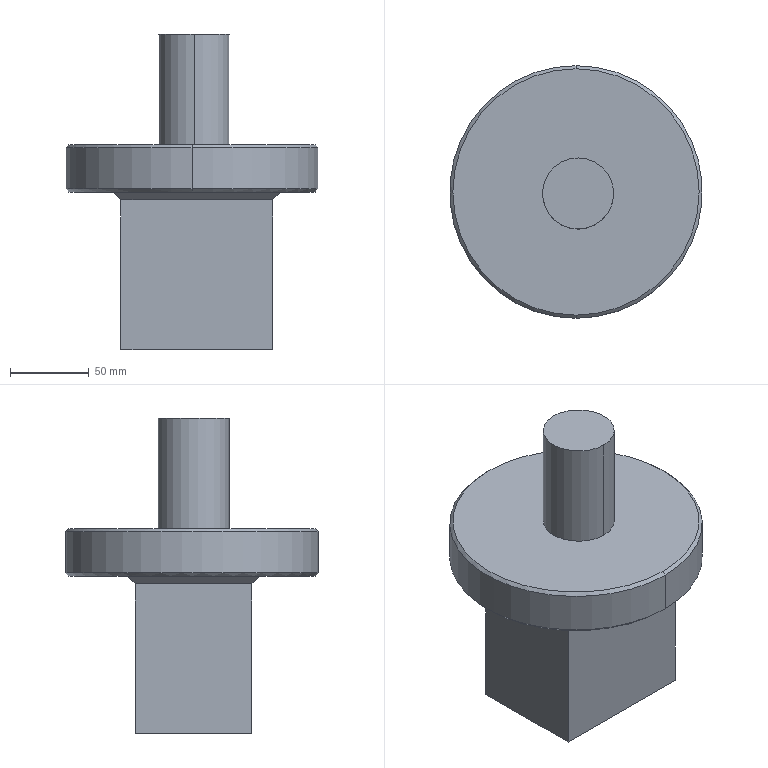Component | SolidWorks | PressureHead-1 | 1 solid | 20 faces | box 160 x 160 x 200 mm | volume 1427339 mm3 | plane 12 | cone 4 | cylinder 4 | commonest cylinder face diameters 45 x2 160 x2
build123d program:
from build123d import *

# Parameters (mm, degrees)
SKETCH1_W           = 80
SKETCH1_H           = 30
SKETCH2_W           = 74
SKETCH2_H           = 96
BOSS_EXTRUDE1_DEPTH = 100
SKETCH3_W           = 22.5
SKETCH3_H           = 70
CHAMFER1_SIZE2      = 2
CHAMFER1_SIZE       = 2
CHAMFER2_SIZE       = 5


with BuildPart() as part:
    # Sketch1 → Revolve1 (revolve)
    with BuildSketch(Plane.XZ.offset(1.405), mode=Mode.PRIVATE) as revolve1_sk:
        with Locations((41.055, 15)):
            Rectangle(SKETCH1_W, SKETCH1_H)
    revolve(revolve1_sk.sketch.rotate(Axis((1.055, -1.405, 30), (0, 0, -1)), 180), axis=Axis((1.055, -1.405, 30), (0, 0, -1)))

    # Sketch2 → Boss-Extrude1 (add)
    with BuildSketch(Plane.XY.offset(30)):
        with Locations((0.05486, 1.595)):
            Rectangle(SKETCH2_W, SKETCH2_H)
    extrude(amount=BOSS_EXTRUDE1_DEPTH)

    # Sketch3 → Revolve2 (revolve)
    with BuildSketch(Plane.XZ, mode=Mode.PRIVATE) as revolve2_sk:
        with Locations((11.25, -35)):
            Rectangle(SKETCH3_W, SKETCH3_H)
    revolve(revolve2_sk.sketch.rotate(Axis((0, 0, 0), (0, 0, -1)), 180), axis=Axis((0, 0, 0), (0, 0, -1)))

    # Chamfer1
    chamfer1_edges = [part.edges().sort_by_distance(p)[0] for p in [
        (81.055, -1.405, 0),
        (81.055, -1.405, 30),
    ]]
    chamfer(chamfer1_edges, length=CHAMFER1_SIZE, length2=CHAMFER1_SIZE2)

    # Chamfer2
    chamfer2_edges = [part.edges().sort_by_distance(p)[0] for p in [
        (-36.945, 1.595, 30),
        (0.05486, -46.405, 30),
        (37.055, 1.595, 30),
        (0.05486, 49.595, 30),
    ]]
    chamfer(chamfer2_edges, length=CHAMFER2_SIZE)


solid = part.part

# Placed as in the assembly
solid = solid.moved(Location((-502.332, 847.548, 384.663), (180, 0, -90)))
STEP:
#1=COLOUR_RGB('',0.7922,0.8196,0.9333);
#2=FILL_AREA_STYLE_COLOUR('',#1);
#3=FILL_AREA_STYLE('',(#2));
#4=SURFACE_STYLE_FILL_AREA(#3);
#5=SURFACE_SIDE_STYLE('',(#4));
#6=SURFACE_STYLE_USAGE(.BOTH.,#5);
#7=PRESENTATION_STYLE_ASSIGNMENT((#6));
#8=CARTESIAN_POINT('',(-19.832,36.48,13.963));
#9=VERTEX_POINT('',#8);
#10=CARTESIAN_POINT('',(-19.832,30.339,13.963));
#11=VERTEX_POINT('',#10);
#12=CARTESIAN_POINT('',(-19.832,33.41,13.963));
#13=DIRECTION('',(0.,0.,-1.));
#14=DIRECTION('',(0.,1.,0.));
#15=AXIS2_PLACEMENT_3D('',#12,#13,#14);
#16=CIRCLE('',#15,3.071);
#17=EDGE_CURVE('',#9,#11,#16,.T.);
#18=ORIENTED_EDGE('',*,*,#17,.F.);
#19=CARTESIAN_POINT('',(-19.832,36.559,14.042));
#20=VERTEX_POINT('',#19);
#21=CARTESIAN_POINT('',(-19.832,36.559,14.042));
#22=DIRECTION('',(0.,0.7071,0.7071));
#23=VECTOR('',#22,39.37);
#24=LINE('',#21,#23);
#25=EDGE_CURVE('',#9,#20,#24,.T.);
#26=ORIENTED_EDGE('',*,*,#25,.T.);
#27=CARTESIAN_POINT('',(-19.832,30.26,14.042));
#28=VERTEX_POINT('',#27);
#29=CARTESIAN_POINT('',(-19.832,33.41,14.042));
#30=DIRECTION('',(0.,0.,1.));
#31=DIRECTION('',(0.,1.,0.));
#32=AXIS2_PLACEMENT_3D('',#29,#30,#31);
#33=CIRCLE('',#32,3.15);
#34=EDGE_CURVE('',#28,#20,#33,.T.);
#35=ORIENTED_EDGE('',*,*,#34,.F.);
#36=CARTESIAN_POINT('',(-19.832,30.26,14.042));
#37=DIRECTION('',(0.,-0.7071,0.7071));
#38=VECTOR('',#37,39.37);
#39=LINE('',#36,#38);
#40=EDGE_CURVE('',#11,#28,#39,.T.);
#41=ORIENTED_EDGE('',*,*,#40,.F.);
#42=EDGE_LOOP('',(#18,#26,#35,#41));
#43=FACE_OUTER_BOUND('',#42,.T.);
#44=CARTESIAN_POINT('',(-19.832,33.41,14.042));
#45=DIRECTION('',(0.,0.,1.));
#46=DIRECTION('',(0.,-1.,0.));
#47=AXIS2_PLACEMENT_3D('',#44,#45,#46);
#48=CONICAL_SURFACE('',#47,3.15,0.7854);
#49=ADVANCED_FACE('',(#43),#48,.T.);
#50=CARTESIAN_POINT('',(-19.832,30.339,15.144));
#51=VERTEX_POINT('',#50);
#52=CARTESIAN_POINT('',(-19.832,36.48,15.144));
#53=VERTEX_POINT('',#52);
#54=CARTESIAN_POINT('',(-19.832,33.41,15.144));
#55=DIRECTION('',(0.,0.,1.));
#56=DIRECTION('',(0.,-1.,0.));
#57=AXIS2_PLACEMENT_3D('',#54,#55,#56);
#58=CIRCLE('',#57,3.071);
#59=EDGE_CURVE('',#51,#53,#58,.T.);
#60=ORIENTED_EDGE('',*,*,#59,.F.);
#61=CARTESIAN_POINT('',(-19.832,30.26,15.065));
#62=VERTEX_POINT('',#61);
#63=CARTESIAN_POINT('',(-19.832,30.339,15.144));
#64=DIRECTION('',(0.,-0.7071,-0.7071));
#65=VECTOR('',#64,39.37);
#66=LINE('',#63,#65);
#67=EDGE_CURVE('',#51,#62,#66,.T.);
#68=ORIENTED_EDGE('',*,*,#67,.T.);
#69=CARTESIAN_POINT('',(-19.832,36.559,15.065));
#70=VERTEX_POINT('',#69);
#71=CARTESIAN_POINT('',(-19.832,33.41,15.065));
#72=DIRECTION('',(0.,0.,-1.));
#73=DIRECTION('',(0.,-1.,0.));
#74=AXIS2_PLACEMENT_3D('',#71,#72,#73);
#75=CIRCLE('',#74,3.15);
#76=EDGE_CURVE('',#70,#62,#75,.T.);
#77=ORIENTED_EDGE('',*,*,#76,.F.);
#78=CARTESIAN_POINT('',(-19.832,36.48,15.144));
#79=DIRECTION('',(0.,0.7071,-0.7071));
#80=VECTOR('',#79,39.37);
#81=LINE('',#78,#80);
#82=EDGE_CURVE('',#53,#70,#81,.T.);
#83=ORIENTED_EDGE('',*,*,#82,.F.);
#84=EDGE_LOOP('',(#60,#68,#77,#83));
#85=FACE_OUTER_BOUND('',#84,.T.);
#86=CARTESIAN_POINT('',(-19.832,33.41,15.144));
#87=DIRECTION('',(0.,0.,-1.));
#88=DIRECTION('',(0.,1.,0.));
#89=AXIS2_PLACEMENT_3D('',#86,#87,#88);
#90=CONICAL_SURFACE('',#89,3.071,0.7854);
#91=ADVANCED_FACE('',(#85),#90,.T.);
#92=CARTESIAN_POINT('',(-19.777,32.482,15.144));
#93=VERTEX_POINT('',#92);
#94=CARTESIAN_POINT('',(-19.777,34.254,15.144));
#95=VERTEX_POINT('',#94);
#96=CARTESIAN_POINT('',(-19.777,33.368,15.144));
#97=DIRECTION('',(0.,0.,1.));
#98=DIRECTION('',(0.,-1.,0.));
#99=AXIS2_PLACEMENT_3D('',#96,#97,#98);
#100=CIRCLE('',#99,0.8858);
#101=EDGE_CURVE('',#93,#95,#100,.T.);
#102=ORIENTED_EDGE('',*,*,#101,.T.);
#103=CARTESIAN_POINT('',(-19.777,34.254,17.9));
#104=VERTEX_POINT('',#103);
#105=CARTESIAN_POINT('',(-19.777,34.254,15.144));
#106=DIRECTION('',(0.,0.,1.));
#107=VECTOR('',#106,39.37);
#108=LINE('',#105,#107);
#109=EDGE_CURVE('',#95,#104,#108,.T.);
#110=ORIENTED_EDGE('',*,*,#109,.T.);
#111=CARTESIAN_POINT('',(-19.777,32.482,17.9));
#112=VERTEX_POINT('',#111);
#113=CARTESIAN_POINT('',(-19.777,33.368,17.9));
#114=DIRECTION('',(0.,0.,1.));
#115=DIRECTION('',(0.,-1.,0.));
#116=AXIS2_PLACEMENT_3D('',#113,#114,#115);
#117=CIRCLE('',#116,0.8858);
#118=EDGE_CURVE('',#112,#104,#117,.T.);
#119=ORIENTED_EDGE('',*,*,#118,.F.);
#120=CARTESIAN_POINT('',(-19.777,32.482,15.144));
#121=DIRECTION('',(0.,0.,1.));
#122=VECTOR('',#121,39.37);
#123=LINE('',#120,#122);
#124=EDGE_CURVE('',#93,#112,#123,.T.);
#125=ORIENTED_EDGE('',*,*,#124,.F.);
#126=EDGE_LOOP('',(#102,#110,#119,#125));
#127=FACE_OUTER_BOUND('',#126,.T.);
#128=CARTESIAN_POINT('',(-19.777,33.368,15.144));
#129=DIRECTION('',(0.,0.,1.));
#130=DIRECTION('',(0.,-1.,0.));
#131=AXIS2_PLACEMENT_3D('',#128,#129,#130);
#132=CYLINDRICAL_SURFACE('',#131,0.8858);
#133=ADVANCED_FACE('',(#127),#132,.T.);
#134=ORIENTED_EDGE('',*,*,#34,.T.);
#135=CARTESIAN_POINT('',(-19.832,36.559,13.963));
#136=DIRECTION('',(0.,0.,1.));
#137=VECTOR('',#136,39.37);
#138=LINE('',#135,#137);
#139=EDGE_CURVE('',#20,#70,#138,.T.);
#140=ORIENTED_EDGE('',*,*,#139,.T.);
#141=ORIENTED_EDGE('',*,*,#76,.T.);
#142=CARTESIAN_POINT('',(-19.832,30.26,13.963));
#143=DIRECTION('',(0.,0.,1.));
#144=VECTOR('',#143,39.37);
#145=LINE('',#142,#144);
#146=EDGE_CURVE('',#28,#62,#145,.T.);
#147=ORIENTED_EDGE('',*,*,#146,.F.);
#148=EDGE_LOOP('',(#134,#140,#141,#147));
#149=FACE_OUTER_BOUND('',#148,.T.);
#150=CARTESIAN_POINT('',(-19.832,33.41,13.963));
#151=DIRECTION('',(0.,0.,1.));
#152=DIRECTION('',(0.,-1.,0.));
#153=AXIS2_PLACEMENT_3D('',#150,#151,#152);
#154=CYLINDRICAL_SURFACE('',#153,3.15);
#155=ADVANCED_FACE('',(#149),#154,.T.);
#156=ORIENTED_EDGE('',*,*,#139,.F.);
#157=CARTESIAN_POINT('',(-19.832,33.41,14.042));
#158=DIRECTION('',(0.,0.,1.));
#159=DIRECTION('',(0.,1.,0.));
#160=AXIS2_PLACEMENT_3D('',#157,#158,#159);
#161=CIRCLE('',#160,3.15);
#162=EDGE_CURVE('',#20,#28,#161,.T.);
#163=ORIENTED_EDGE('',*,*,#162,.T.);
#164=ORIENTED_EDGE('',*,*,#146,.T.);
#165=CARTESIAN_POINT('',(-19.832,33.41,15.065));
#166=DIRECTION('',(0.,0.,-1.));
#167=DIRECTION('',(0.,-1.,0.));
#168=AXIS2_PLACEMENT_3D('',#165,#166,#167);
#169=CIRCLE('',#168,3.15);
#170=EDGE_CURVE('',#62,#70,#169,.T.);
#171=ORIENTED_EDGE('',*,*,#170,.T.);
#172=EDGE_LOOP('',(#156,#163,#164,#171));
#173=FACE_OUTER_BOUND('',#172,.T.);
#174=CARTESIAN_POINT('',(-19.832,33.41,13.963));
#175=DIRECTION('',(0.,0.,1.));
#176=DIRECTION('',(0.,-1.,0.));
#177=AXIS2_PLACEMENT_3D('',#174,#175,#176);
#178=CYLINDRICAL_SURFACE('',#177,3.15);
#179=ADVANCED_FACE('',(#173),#178,.T.);
#180=CARTESIAN_POINT('',(-21.801,35.024,13.963));
#181=VERTEX_POINT('',#180);
#182=CARTESIAN_POINT('',(-21.801,31.717,13.963));
#183=VERTEX_POINT('',#182);
#184=CARTESIAN_POINT('',(-21.801,36.559,13.963));
#185=DIRECTION('',(0.,-1.,0.));
#186=VECTOR('',#185,39.37);
#187=LINE('',#184,#186);
#188=EDGE_CURVE('',#181,#183,#187,.T.);
#189=ORIENTED_EDGE('',*,*,#188,.T.);
#190=CARTESIAN_POINT('',(-17.627,31.717,13.963));
#191=VERTEX_POINT('',#190);
#192=CARTESIAN_POINT('',(-19.832,31.717,13.963));
#193=DIRECTION('',(1.,0.,0.));
#194=VECTOR('',#193,39.37);
#195=LINE('',#192,#194);
#196=EDGE_CURVE('',#183,#191,#195,.T.);
#197=ORIENTED_EDGE('',*,*,#196,.T.);
#198=CARTESIAN_POINT('',(-17.627,35.024,13.963));
#199=VERTEX_POINT('',#198);
#200=CARTESIAN_POINT('',(-17.627,36.559,13.963));
#201=DIRECTION('',(0.,1.,0.));
#202=VECTOR('',#201,39.37);
#203=LINE('',#200,#202);
#204=EDGE_CURVE('',#191,#199,#203,.T.);
#205=ORIENTED_EDGE('',*,*,#204,.T.);
#206=CARTESIAN_POINT('',(-19.832,35.024,13.963));
#207=DIRECTION('',(-1.,0.,0.));
#208=VECTOR('',#207,39.37);
#209=LINE('',#206,#208);
#210=EDGE_CURVE('',#199,#181,#209,.T.);
#211=ORIENTED_EDGE('',*,*,#210,.T.);
#212=EDGE_LOOP('',(#189,#197,#205,#211));
#213=FACE_BOUND('',#212,.T.);
#214=CARTESIAN_POINT('',(-19.832,33.41,13.963));
#215=DIRECTION('',(0.,0.,-1.));
#216=DIRECTION('',(0.,1.,0.));
#217=AXIS2_PLACEMENT_3D('',#214,#215,#216);
#218=CIRCLE('',#217,3.071);
#219=EDGE_CURVE('',#11,#9,#218,.T.);
#220=ORIENTED_EDGE('',*,*,#219,.T.);
#221=ORIENTED_EDGE('',*,*,#17,.T.);
#222=EDGE_LOOP('',(#220,#221));
#223=FACE_OUTER_BOUND('',#222,.T.);
#224=CARTESIAN_POINT('',(-19.832,36.559,13.963));
#225=DIRECTION('',(0.,0.,-1.));
#226=DIRECTION('',(0.,1.,0.));
#227=AXIS2_PLACEMENT_3D('',#224,#225,#226);
#228=PLANE('',#227);
#229=ADVANCED_FACE('',(#213,#223),#228,.T.);
#230=CARTESIAN_POINT('',(-19.832,33.41,15.144));
#231=DIRECTION('',(0.,0.,1.));
#232=DIRECTION('',(0.,-1.,0.));
#233=AXIS2_PLACEMENT_3D('',#230,#231,#232);
#234=CIRCLE('',#233,3.071);
#235=EDGE_CURVE('',#53,#51,#234,.T.);
#236=ORIENTED_EDGE('',*,*,#235,.T.);
#237=ORIENTED_EDGE('',*,*,#59,.T.);
#238=EDGE_LOOP('',(#236,#237));
#239=FACE_OUTER_BOUND('',#238,.T.);
#240=ORIENTED_EDGE('',*,*,#101,.F.);
#241=CARTESIAN_POINT('',(-19.777,33.368,15.144));
#242=DIRECTION('',(0.,0.,1.));
#243=DIRECTION('',(0.,-1.,0.));
#244=AXIS2_PLACEMENT_3D('',#241,#242,#243);
#245=CIRCLE('',#244,0.8858);
#246=EDGE_CURVE('',#95,#93,#245,.T.);
#247=ORIENTED_EDGE('',*,*,#246,.F.);
#248=EDGE_LOOP('',(#240,#247));
#249=FACE_BOUND('',#248,.T.);
#250=CARTESIAN_POINT('',(-19.832,33.41,15.144));
#251=DIRECTION('',(0.,0.,1.));
#252=DIRECTION('',(0.,-1.,0.));
#253=AXIS2_PLACEMENT_3D('',#250,#251,#252);
#254=PLANE('',#253);
#255=ADVANCED_FACE('',(#239,#249),#254,.T.);
#256=CARTESIAN_POINT('',(-17.824,31.913,10.026));
#257=VERTEX_POINT('',#256);
#258=CARTESIAN_POINT('',(-17.824,31.913,13.766));
#259=VERTEX_POINT('',#258);
#260=CARTESIAN_POINT('',(-17.824,31.913,10.026));
#261=DIRECTION('',(0.,0.,1.));
#262=VECTOR('',#261,39.37);
#263=LINE('',#260,#262);
#264=EDGE_CURVE('',#257,#259,#263,.T.);
#265=ORIENTED_EDGE('',*,*,#264,.T.);
#266=CARTESIAN_POINT('',(-21.604,31.913,13.766));
#267=VERTEX_POINT('',#266);
#268=CARTESIAN_POINT('',(-21.604,31.913,13.766));
#269=DIRECTION('',(-1.,0.,0.));
#270=VECTOR('',#269,39.37);
#271=LINE('',#268,#270);
#272=EDGE_CURVE('',#259,#267,#271,.T.);
#273=ORIENTED_EDGE('',*,*,#272,.T.);
#274=CARTESIAN_POINT('',(-21.604,31.913,10.026));
#275=VERTEX_POINT('',#274);
#276=CARTESIAN_POINT('',(-21.604,31.913,10.026));
#277=DIRECTION('',(0.,0.,1.));
#278=VECTOR('',#277,39.37);
#279=LINE('',#276,#278);
#280=EDGE_CURVE('',#275,#267,#279,.T.);
#281=ORIENTED_EDGE('',*,*,#280,.F.);
#282=CARTESIAN_POINT('',(-21.604,31.913,10.026));
#283=DIRECTION('',(-1.,0.,0.));
#284=VECTOR('',#283,39.37);
#285=LINE('',#282,#284);
#286=EDGE_CURVE('',#257,#275,#285,.T.);
#287=ORIENTED_EDGE('',*,*,#286,.F.);
#288=EDGE_LOOP('',(#265,#273,#281,#287));
#289=FACE_OUTER_BOUND('',#288,.T.);
#290=CARTESIAN_POINT('',(-21.604,31.913,10.026));
#291=DIRECTION('',(0.,1.,0.));
#292=DIRECTION('',(0.,0.,1.));
#293=AXIS2_PLACEMENT_3D('',#290,#291,#292);
#294=PLANE('',#293);
#295=ADVANCED_FACE('',(#289),#294,.F.);
#296=ORIENTED_EDGE('',*,*,#280,.T.);
#297=CARTESIAN_POINT('',(-21.604,34.827,13.766));
#298=VERTEX_POINT('',#297);
#299=CARTESIAN_POINT('',(-21.604,34.827,13.766));
#300=DIRECTION('',(0.,1.,0.));
#301=VECTOR('',#300,39.37);
#302=LINE('',#299,#301);
#303=EDGE_CURVE('',#267,#298,#302,.T.);
#304=ORIENTED_EDGE('',*,*,#303,.T.);
#305=CARTESIAN_POINT('',(-21.604,34.827,10.026));
#306=VERTEX_POINT('',#305);
#307=CARTESIAN_POINT('',(-21.604,34.827,10.026));
#308=DIRECTION('',(0.,0.,1.));
#309=VECTOR('',#308,39.37);
#310=LINE('',#307,#309);
#311=EDGE_CURVE('',#306,#298,#310,.T.);
#312=ORIENTED_EDGE('',*,*,#311,.F.);
#313=CARTESIAN_POINT('',(-21.604,34.827,10.026));
#314=DIRECTION('',(0.,1.,0.));
#315=VECTOR('',#314,39.37);
#316=LINE('',#313,#315);
#317=EDGE_CURVE('',#275,#306,#316,.T.);
#318=ORIENTED_EDGE('',*,*,#317,.F.);
#319=EDGE_LOOP('',(#296,#304,#312,#318));
#320=FACE_OUTER_BOUND('',#319,.T.);
#321=CARTESIAN_POINT('',(-21.604,34.827,10.026));
#322=DIRECTION('',(1.,0.,0.));
#323=DIRECTION('',(0.,0.,-1.));
#324=AXIS2_PLACEMENT_3D('',#321,#322,#323);
#325=PLANE('',#324);
#326=ADVANCED_FACE('',(#320),#325,.F.);
#327=ORIENTED_EDGE('',*,*,#311,.T.);
#328=CARTESIAN_POINT('',(-17.824,34.827,13.766));
#329=VERTEX_POINT('',#328);
#330=CARTESIAN_POINT('',(-17.824,34.827,13.766));
#331=DIRECTION('',(1.,0.,0.));
#332=VECTOR('',#331,39.37);
#333=LINE('',#330,#332);
#334=EDGE_CURVE('',#298,#329,#333,.T.);
#335=ORIENTED_EDGE('',*,*,#334,.T.);
#336=CARTESIAN_POINT('',(-17.824,34.827,10.026));
#337=VERTEX_POINT('',#336);
#338=CARTESIAN_POINT('',(-17.824,34.827,10.026));
#339=DIRECTION('',(0.,0.,1.));
#340=VECTOR('',#339,39.37);
#341=LINE('',#338,#340);
#342=EDGE_CURVE('',#337,#329,#341,.T.);
#343=ORIENTED_EDGE('',*,*,#342,.F.);
#344=CARTESIAN_POINT('',(-17.824,34.827,10.026));
#345=DIRECTION('',(1.,0.,0.));
#346=VECTOR('',#345,39.37);
#347=LINE('',#344,#346);
#348=EDGE_CURVE('',#306,#337,#347,.T.);
#349=ORIENTED_EDGE('',*,*,#348,.F.);
#350=EDGE_LOOP('',(#327,#335,#343,#349));
#351=FACE_OUTER_BOUND('',#350,.T.);
#352=CARTESIAN_POINT('',(-17.824,34.827,10.026));
#353=DIRECTION('',(0.,-1.,0.));
#354=DIRECTION('',(0.,0.,-1.));
#355=AXIS2_PLACEMENT_3D('',#352,#353,#354);
#356=PLANE('',#355);
#357=ADVANCED_FACE('',(#351),#356,.F.);
#358=ORIENTED_EDGE('',*,*,#342,.T.);
#359=CARTESIAN_POINT('',(-17.824,31.913,13.766));
#360=DIRECTION('',(0.,-1.,0.));
#361=VECTOR('',#360,39.37);
#362=LINE('',#359,#361);
#363=EDGE_CURVE('',#329,#259,#362,.T.);
#364=ORIENTED_EDGE('',*,*,#363,.T.);
#365=ORIENTED_EDGE('',*,*,#264,.F.);
#366=CARTESIAN_POINT('',(-17.824,31.913,10.026));
#367=DIRECTION('',(0.,-1.,0.));
#368=VECTOR('',#367,39.37);
#369=LINE('',#366,#368);
#370=EDGE_CURVE('',#337,#257,#369,.T.);
#371=ORIENTED_EDGE('',*,*,#370,.F.);
#372=EDGE_LOOP('',(#358,#364,#365,#371));
#373=FACE_OUTER_BOUND('',#372,.T.);
#374=CARTESIAN_POINT('',(-17.824,31.913,10.026));
#375=DIRECTION('',(-1.,0.,0.));
#376=DIRECTION('',(0.,0.,1.));
#377=AXIS2_PLACEMENT_3D('',#374,#375,#376);
#378=PLANE('',#377);
#379=ADVANCED_FACE('',(#373),#378,.F.);
#380=ORIENTED_EDGE('',*,*,#286,.T.);
#381=ORIENTED_EDGE('',*,*,#317,.T.);
#382=ORIENTED_EDGE('',*,*,#348,.T.);
#383=ORIENTED_EDGE('',*,*,#370,.T.);
#384=EDGE_LOOP('',(#380,#381,#382,#383));
#385=FACE_OUTER_BOUND('',#384,.T.);
#386=CARTESIAN_POINT('',(-19.777,33.368,10.026));
#387=DIRECTION('',(0.,0.,1.));
#388=DIRECTION('',(0.,-1.,0.));
#389=AXIS2_PLACEMENT_3D('',#386,#387,#388);
#390=PLANE('',#389);
#391=ADVANCED_FACE('',(#385),#390,.F.);
#392=ORIENTED_EDGE('',*,*,#109,.F.);
#393=ORIENTED_EDGE('',*,*,#246,.T.);
#394=ORIENTED_EDGE('',*,*,#124,.T.);
#395=CARTESIAN_POINT('',(-19.777,33.368,17.9));
#396=DIRECTION('',(0.,0.,1.));
#397=DIRECTION('',(0.,-1.,0.));
#398=AXIS2_PLACEMENT_3D('',#395,#396,#397);
#399=CIRCLE('',#398,0.8858);
#400=EDGE_CURVE('',#104,#112,#399,.T.);
#401=ORIENTED_EDGE('',*,*,#400,.F.);
#402=EDGE_LOOP('',(#392,#393,#394,#401));
#403=FACE_OUTER_BOUND('',#402,.T.);
#404=CARTESIAN_POINT('',(-19.777,33.368,15.144));
#405=DIRECTION('',(0.,0.,1.));
#406=DIRECTION('',(0.,-1.,0.));
#407=AXIS2_PLACEMENT_3D('',#404,#405,#406);
#408=CYLINDRICAL_SURFACE('',#407,0.8858);
#409=ADVANCED_FACE('',(#403),#408,.T.);
#410=ORIENTED_EDGE('',*,*,#118,.T.);
#411=ORIENTED_EDGE('',*,*,#400,.T.);
#412=EDGE_LOOP('',(#410,#411));
#413=FACE_OUTER_BOUND('',#412,.T.);
#414=CARTESIAN_POINT('',(-19.777,33.368,17.9));
#415=DIRECTION('',(0.,0.,1.));
#416=DIRECTION('',(0.,-1.,0.));
#417=AXIS2_PLACEMENT_3D('',#414,#415,#416);
#418=PLANE('',#417);
#419=ADVANCED_FACE('',(#413),#418,.T.);
#420=ORIENTED_EDGE('',*,*,#67,.F.);
#421=ORIENTED_EDGE('',*,*,#235,.F.);
#422=ORIENTED_EDGE('',*,*,#82,.T.);
#423=ORIENTED_EDGE('',*,*,#170,.F.);
#424=EDGE_LOOP('',(#420,#421,#422,#423));
#425=FACE_OUTER_BOUND('',#424,.T.);
#426=CARTESIAN_POINT('',(-19.832,33.41,15.144));
#427=DIRECTION('',(0.,0.,-1.));
#428=DIRECTION('',(0.,1.,0.));
#429=AXIS2_PLACEMENT_3D('',#426,#427,#428);
#430=CONICAL_SURFACE('',#429,3.071,0.7854);
#431=ADVANCED_FACE('',(#425),#430,.T.);
#432=ORIENTED_EDGE('',*,*,#25,.F.);
#433=ORIENTED_EDGE('',*,*,#219,.F.);
#434=ORIENTED_EDGE('',*,*,#40,.T.);
#435=ORIENTED_EDGE('',*,*,#162,.F.);
#436=EDGE_LOOP('',(#432,#433,#434,#435));
#437=FACE_OUTER_BOUND('',#436,.T.);
#438=CARTESIAN_POINT('',(-19.832,33.41,14.042));
#439=DIRECTION('',(0.,0.,1.));
#440=DIRECTION('',(0.,-1.,0.));
#441=AXIS2_PLACEMENT_3D('',#438,#439,#440);
#442=CONICAL_SURFACE('',#441,3.15,0.7854);
#443=ADVANCED_FACE('',(#437),#442,.T.);
#444=CARTESIAN_POINT('',(-20.344,33.567,12.506));
#445=DIRECTION('',(0.5774,-0.5774,-0.5774));
#446=VECTOR('',#445,39.37);
#447=LINE('',#444,#446);
#448=EDGE_CURVE('',#181,#298,#447,.T.);
#449=ORIENTED_EDGE('',*,*,#448,.F.);
#450=ORIENTED_EDGE('',*,*,#210,.F.);
#451=CARTESIAN_POINT('',(-17.824,34.827,13.766));
#452=DIRECTION('',(0.5774,0.5774,0.5774));
#453=VECTOR('',#452,39.37);
#454=LINE('',#451,#453);
#455=EDGE_CURVE('',#329,#199,#454,.T.);
#456=ORIENTED_EDGE('',*,*,#455,.F.);
#457=ORIENTED_EDGE('',*,*,#334,.F.);
#458=EDGE_LOOP('',(#449,#450,#456,#457));
#459=FACE_OUTER_BOUND('',#458,.T.);
#460=CARTESIAN_POINT('',(-17.824,34.827,13.766));
#461=DIRECTION('',(0.,-0.7071,0.7071));
#462=DIRECTION('',(1.,0.,0.));
#463=AXIS2_PLACEMENT_3D('',#460,#461,#462);
#464=PLANE('',#463);
#465=ADVANCED_FACE('',(#459),#464,.F.);
#466=ORIENTED_EDGE('',*,*,#455,.T.);
#467=ORIENTED_EDGE('',*,*,#204,.F.);
#468=CARTESIAN_POINT('',(-17.824,31.913,13.766));
#469=DIRECTION('',(0.5774,-0.5774,0.5774));
#470=VECTOR('',#469,39.37);
#471=LINE('',#468,#470);
#472=EDGE_CURVE('',#259,#191,#471,.T.);
#473=ORIENTED_EDGE('',*,*,#472,.F.);
#474=ORIENTED_EDGE('',*,*,#363,.F.);
#475=EDGE_LOOP('',(#466,#467,#473,#474));
#476=FACE_OUTER_BOUND('',#475,.T.);
#477=CARTESIAN_POINT('',(-17.824,31.913,13.766));
#478=DIRECTION('',(-0.7071,0.,0.7071));
#479=DIRECTION('',(0.,-1.,0.));
#480=AXIS2_PLACEMENT_3D('',#477,#478,#479);
#481=PLANE('',#480);
#482=ADVANCED_FACE('',(#476),#481,.F.);
#483=ORIENTED_EDGE('',*,*,#448,.T.);
#484=ORIENTED_EDGE('',*,*,#303,.F.);
#485=CARTESIAN_POINT('',(-20.633,32.885,12.795));
#486=DIRECTION('',(0.5774,0.5774,-0.5774));
#487=VECTOR('',#486,39.37);
#488=LINE('',#485,#487);
#489=EDGE_CURVE('',#183,#267,#488,.T.);
#490=ORIENTED_EDGE('',*,*,#489,.F.);
#491=ORIENTED_EDGE('',*,*,#188,.F.);
#492=EDGE_LOOP('',(#483,#484,#490,#491));
#493=FACE_OUTER_BOUND('',#492,.T.);
#494=CARTESIAN_POINT('',(-21.604,34.827,13.766));
#495=DIRECTION('',(0.7071,0.,0.7071));
#496=DIRECTION('',(0.,1.,0.));
#497=AXIS2_PLACEMENT_3D('',#494,#495,#496);
#498=PLANE('',#497);
#499=ADVANCED_FACE('',(#493),#498,.F.);
#500=ORIENTED_EDGE('',*,*,#472,.T.);
#501=ORIENTED_EDGE('',*,*,#196,.F.);
#502=ORIENTED_EDGE('',*,*,#489,.T.);
#503=ORIENTED_EDGE('',*,*,#272,.F.);
#504=EDGE_LOOP('',(#500,#501,#502,#503));
#505=FACE_OUTER_BOUND('',#504,.T.);
#506=CARTESIAN_POINT('',(-21.604,31.913,13.766));
#507=DIRECTION('',(0.,0.7071,0.7071));
#508=DIRECTION('',(-1.,0.,0.));
#509=AXIS2_PLACEMENT_3D('',#506,#507,#508);
#510=PLANE('',#509);
#511=ADVANCED_FACE('',(#505),#510,.F.);
#512=CLOSED_SHELL('',(#49,#91,#133,#155,#179,#229,#255,#295,#326,#357,#379,#391,#409,#419,#431,#443,#465,#482,#499,#511));
#513=MANIFOLD_SOLID_BREP('',#512);
#514=STYLED_ITEM('',(#7),#513);
#515=PRESENTATION_LAYER_ASSIGNMENT('','',(#514));
#516=CARTESIAN_POINT('',(0.,0.,0.));
#517=DIRECTION('',(0.,0.,1.));
#518=DIRECTION('',(1.,0.,0.));
#519=AXIS2_PLACEMENT_3D('',#516,#517,#518);
#520=(LENGTH_UNIT()NAMED_UNIT(*)SI_UNIT($,.METRE.));
#521=LENGTH_MEASURE_WITH_UNIT(LENGTH_MEASURE(0.0254),#520);
#522=DIMENSIONAL_EXPONENTS(1.,0.,0.,0.,0.,0.,0.);
#523=(CONVERSION_BASED_UNIT('',#521)LENGTH_UNIT()NAMED_UNIT(#522));
#524=UNCERTAINTY_MEASURE_WITH_UNIT(LENGTH_MEASURE(0.00001),#523,'','');
#525=(NAMED_UNIT(*)PLANE_ANGLE_UNIT()SI_UNIT($,.RADIAN.));
#526=(NAMED_UNIT(*)SI_UNIT($,.STERADIAN.)SOLID_ANGLE_UNIT());
#527=(GEOMETRIC_REPRESENTATION_CONTEXT(3)GLOBAL_UNCERTAINTY_ASSIGNED_CONTEXT((#524))GLOBAL_UNIT_ASSIGNED_CONTEXT((#523,#525,#526))REPRESENTATION_CONTEXT('',''));
#528=ADVANCED_BREP_SHAPE_REPRESENTATION('',(#513,#519),#527);
#529=(LENGTH_UNIT()NAMED_UNIT(*)SI_UNIT($,.METRE.));
#530=LENGTH_MEASURE_WITH_UNIT(LENGTH_MEASURE(0.0254),#529);
#531=DIMENSIONAL_EXPONENTS(1.,0.,0.,0.,0.,0.,0.);
#532=(CONVERSION_BASED_UNIT('',#530)LENGTH_UNIT()NAMED_UNIT(#531));
#533=UNCERTAINTY_MEASURE_WITH_UNIT(LENGTH_MEASURE(0.00001),#532,'','');
#534=(NAMED_UNIT(*)PLANE_ANGLE_UNIT()SI_UNIT($,.RADIAN.));
#535=(NAMED_UNIT(*)SI_UNIT($,.STERADIAN.)SOLID_ANGLE_UNIT());
#536=(GEOMETRIC_REPRESENTATION_CONTEXT(3)GLOBAL_UNCERTAINTY_ASSIGNED_CONTEXT((#533))GLOBAL_UNIT_ASSIGNED_CONTEXT((#532,#534,#535))REPRESENTATION_CONTEXT('',''));
#537=MECHANICAL_DESIGN_GEOMETRIC_PRESENTATION_REPRESENTATION('',(#514),#536);